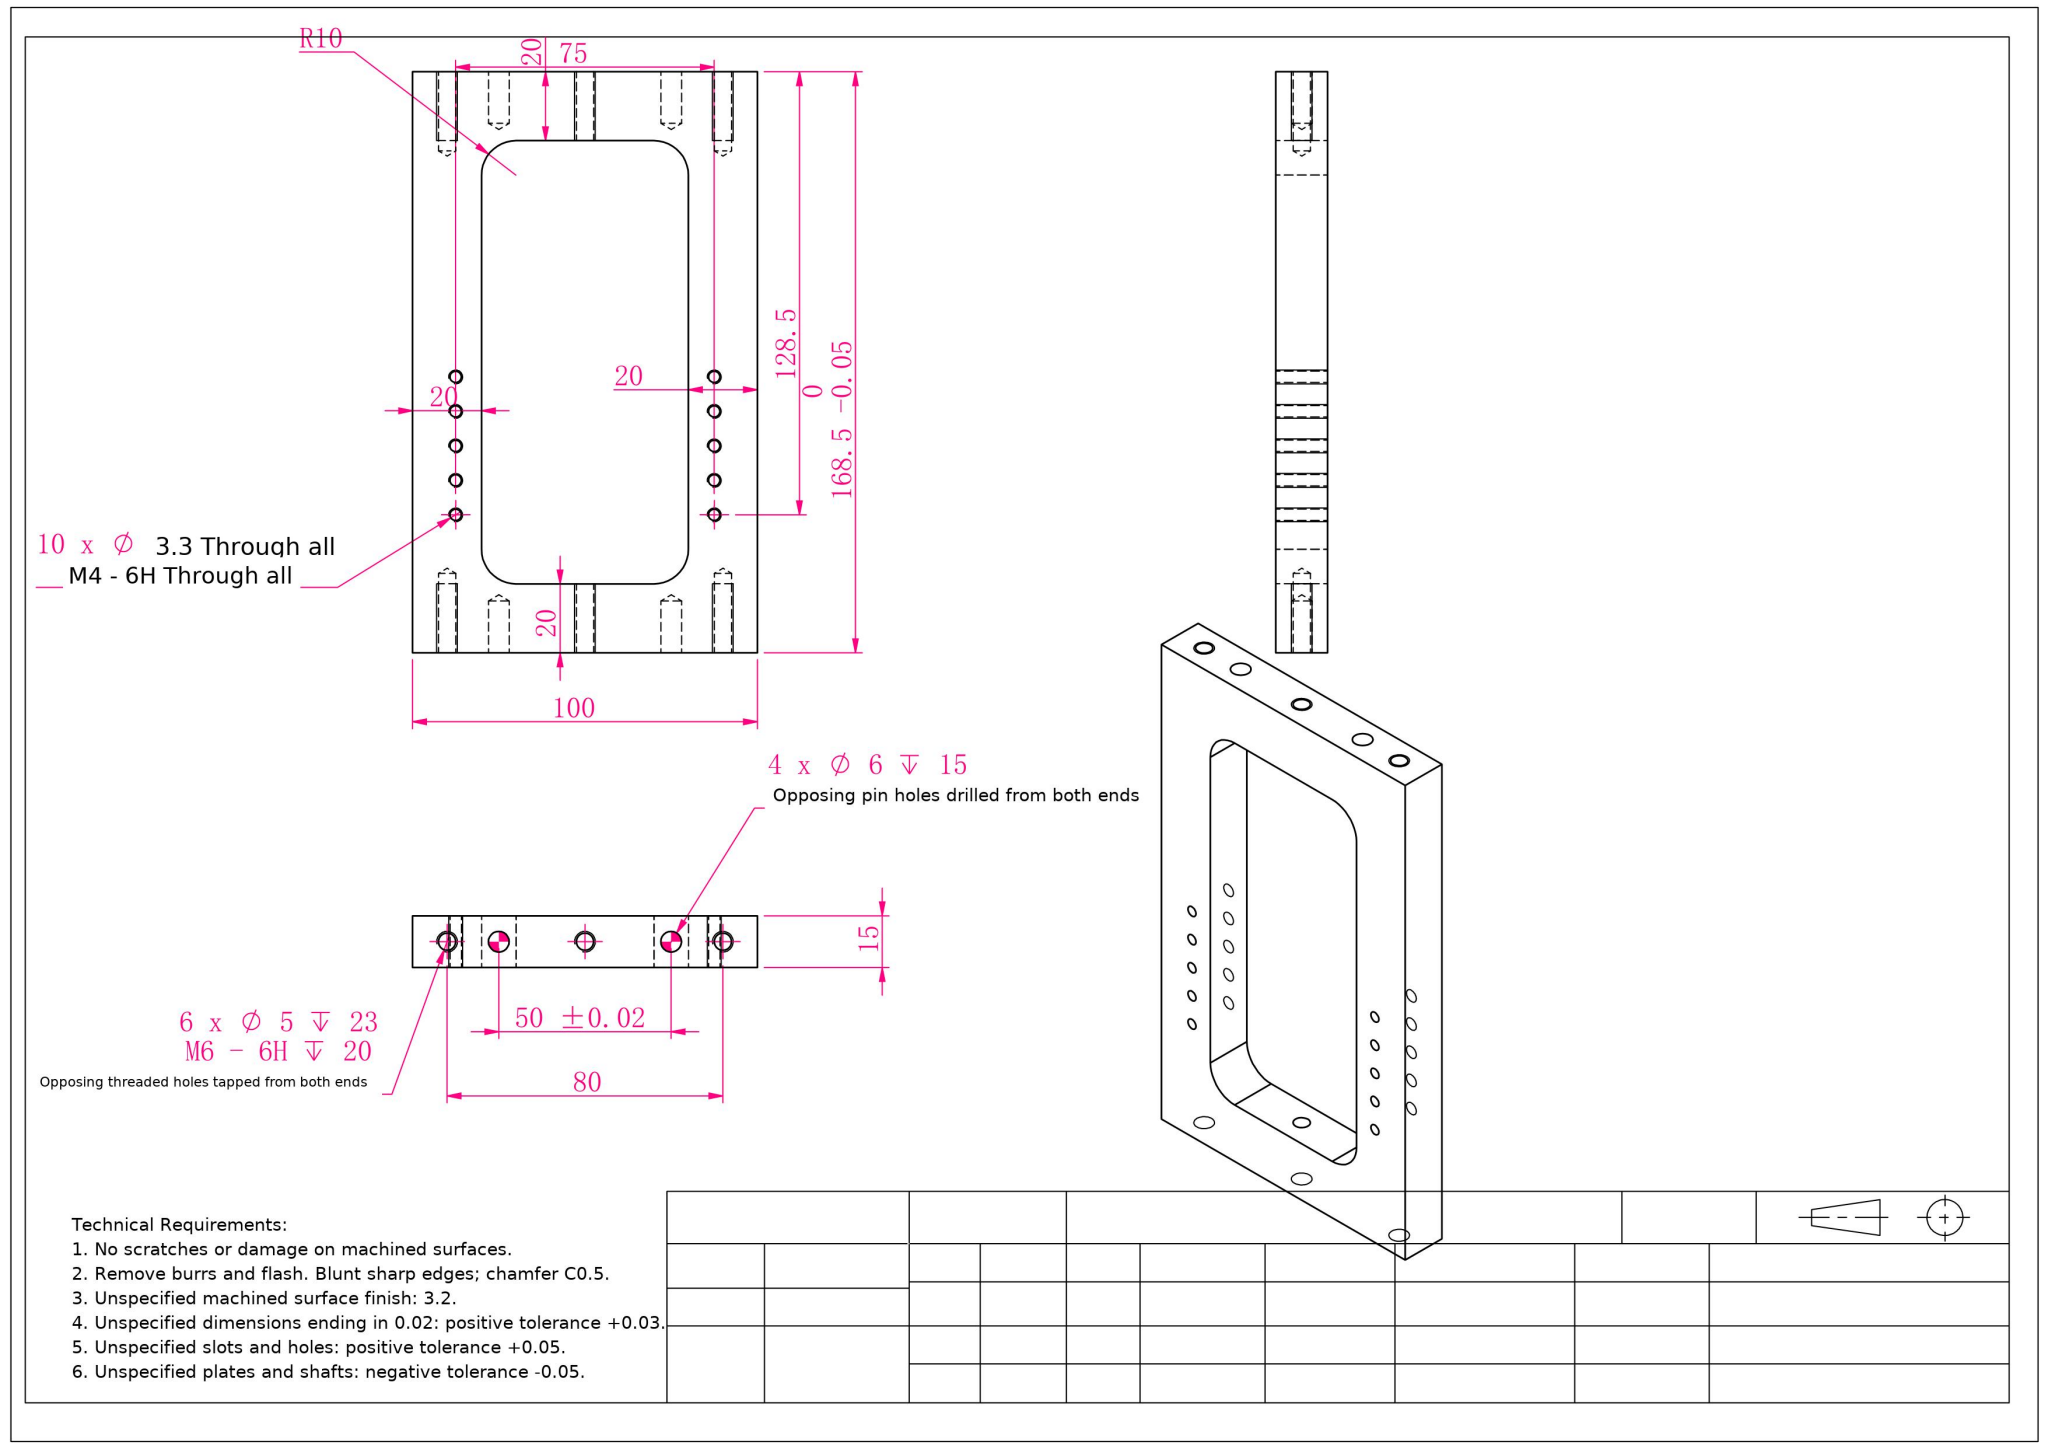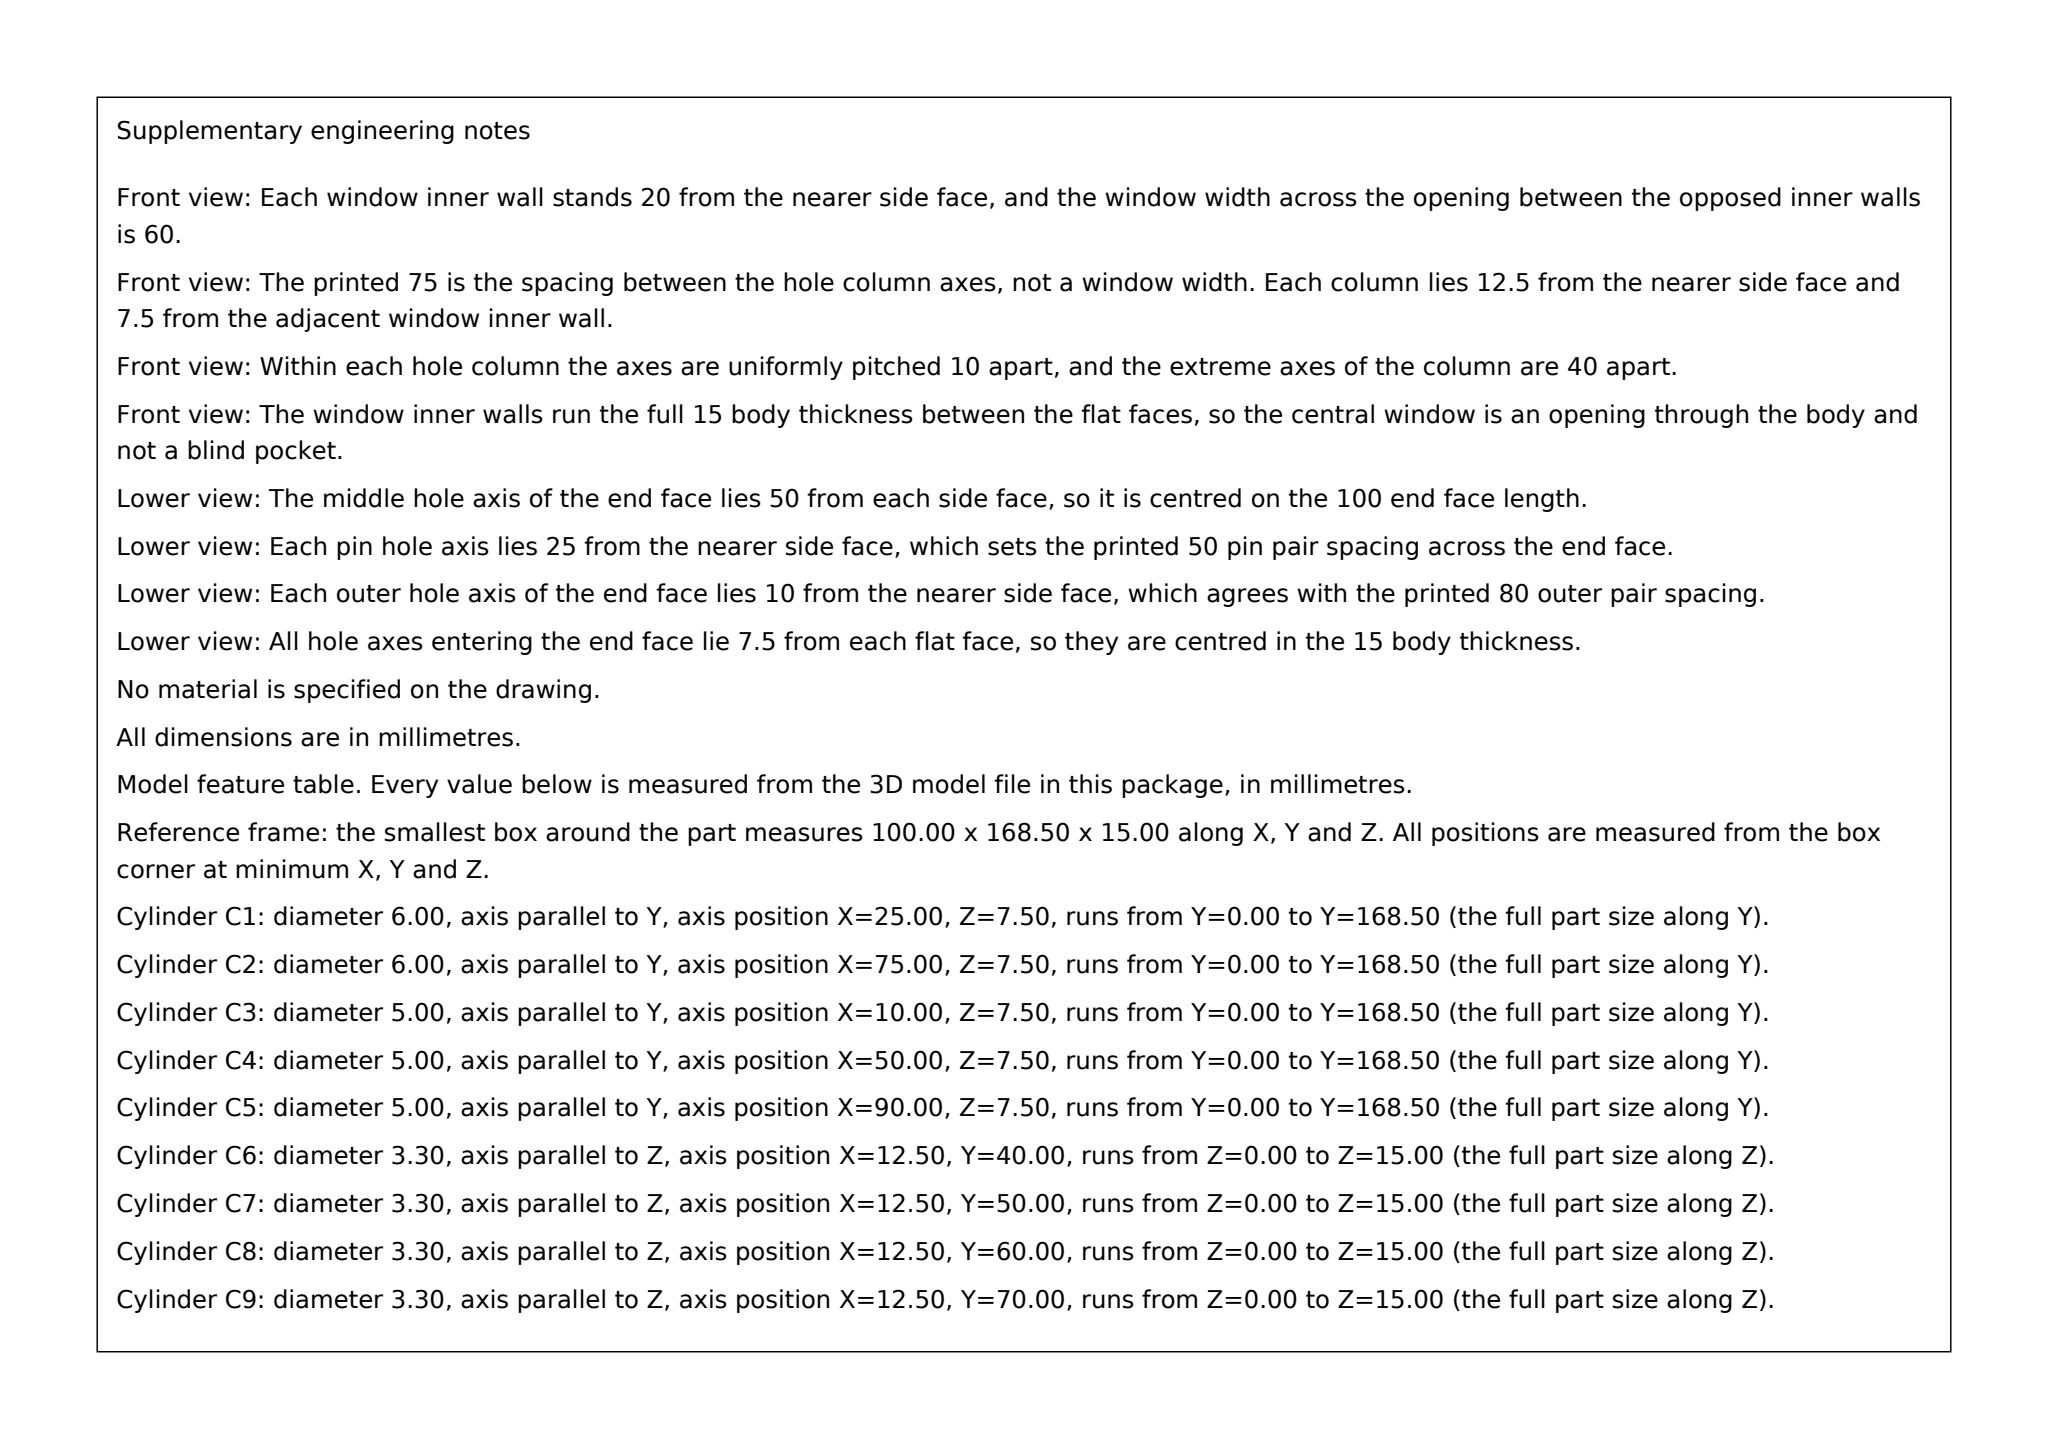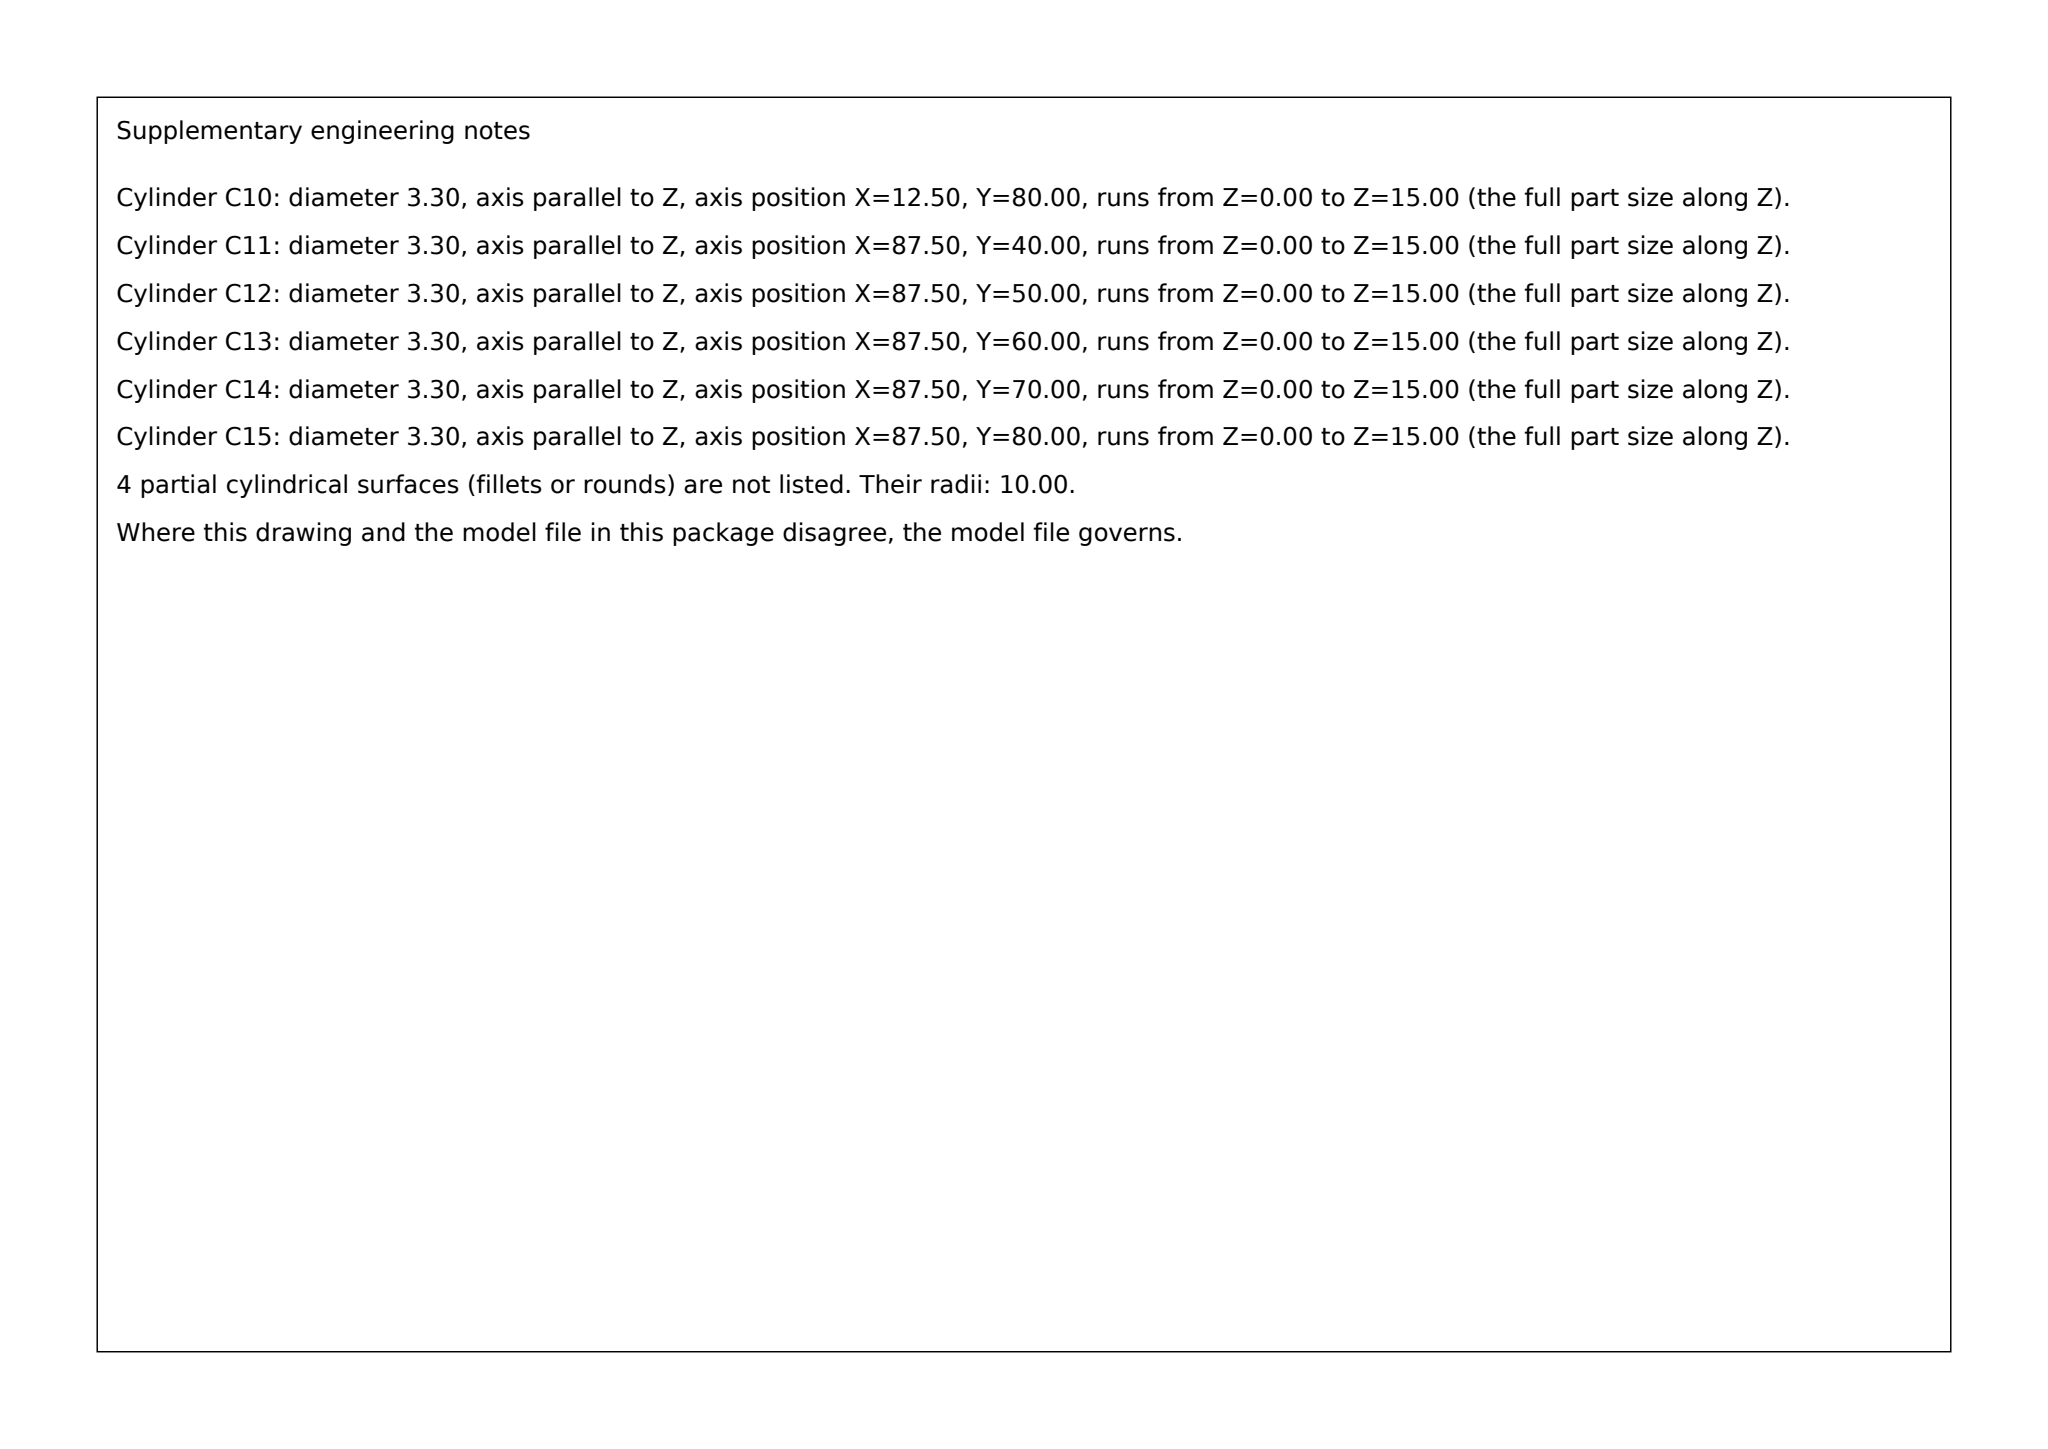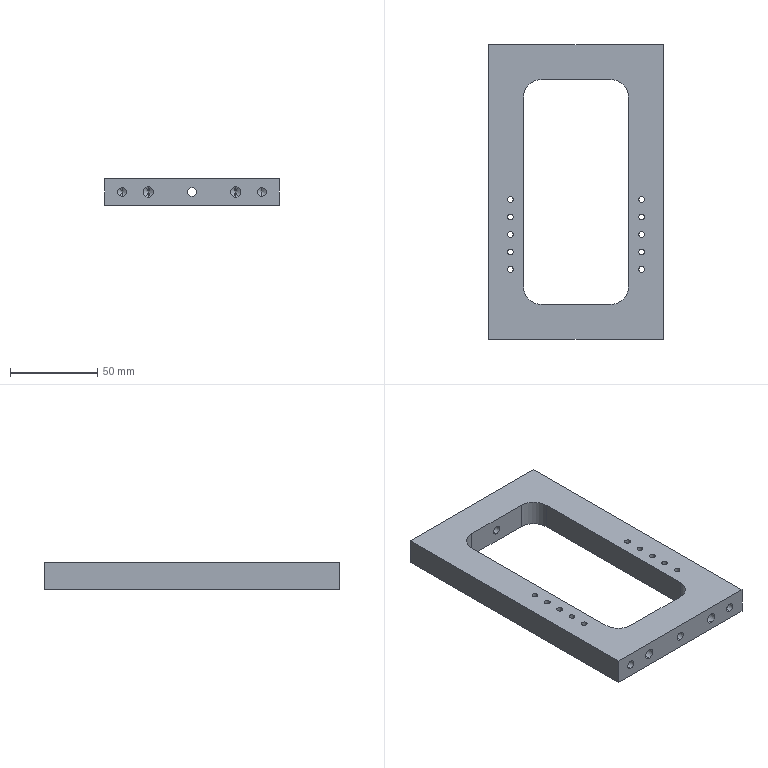Part | SolidWorks | mm | 1 solid | 70 faces | box 100 x 168.5 x 15 mm | volume 132709 mm3 | cylinder 44 | cone 16 | plane 10 | commonest cylinder face diameters 3.3 x20 5 x12 6 x8 20 x4
build123d program:
from build123d import *

# Parameters (mm, degrees)
SKETCH1_W                          = 100
SKETCH1_H                          = 168.5
BOSS_EXTRUDE1_DEPTH                = 7.5
M6_TAPPED_HOLE1_AT_2_COUNT         = 2
M6_TAPPED_HOLE1_AT_2_PITCH         = 40
M6_TAPPED_HOLE1_AT_3_COUNT         = 2
M6_TAPPED_HOLE1_AT_3_PITCH         = 80
SIZE_MM_DOWEL_PIN_HOLE1_AT_2_COUNT = 2
SIZE_MM_DOWEL_PIN_HOLE1_AT_2_PITCH = 50
SKETCH6_W                          = 60
SKETCH6_H                          = 128.5
CUT_EXTRUDE1_DEPTH                 = 100.111
FILLET1_R                          = 10
M4_TAPPED_HOLE1_D                  = 3.3
LPATTERN1_COUNT                    = 5
LPATTERN1_PITCH                    = 10


with BuildPart() as part:
    # Sketch1 → Boss-Extrude1 (new, symmetric)
    with BuildSketch(Plane.XY):
        Rectangle(SKETCH1_W, SKETCH1_H)
    extrude(amount=BOSS_EXTRUDE1_DEPTH, both=True)

    # Sketch3 → M6 Tapped Hole1 (revolve, cut)
    with BuildSketch(Plane(origin=(-40, -84.25, 0), x_dir=(0, 0, -1), z_dir=(1, 0, 0))):
        Polygon((0, 0), (0, 24.502), (2.5, 23), (2.5, 0), align=None)
    m6_tapped_hole1 = revolve(axis=Axis((-40, -90.6, 0), (0, 1, 0)), mode=Mode.SUBTRACT)

    # M6 Tapped Hole1 at 2: M6 Tapped Hole1 ×2
    with Locations(*[(i * M6_TAPPED_HOLE1_AT_2_PITCH, 0, 0) for i in range(1, M6_TAPPED_HOLE1_AT_2_COUNT)]):
        add(m6_tapped_hole1, mode=Mode.SUBTRACT)

    # M6 Tapped Hole1 at 3: M6 Tapped Hole1 ×2
    with Locations(*[(i * M6_TAPPED_HOLE1_AT_3_PITCH, 0, 0) for i in range(1, M6_TAPPED_HOLE1_AT_3_COUNT)]):
        add(m6_tapped_hole1, mode=Mode.SUBTRACT)

    # Sketch5 → Size mm Dowel Pin Hole1 (revolve, cut)
    with BuildSketch(Plane(origin=(-25, -84.25, 0), x_dir=(0, 0, -1), z_dir=(1, 0, 0))):
        Polygon((0, 0), (0, 16.803), (3, 15), (3, 0), align=None)
    size_mm_dowel_pin_hole1 = revolve(axis=Axis((-25, -90.6, 0), (0, 1, 0)), mode=Mode.SUBTRACT)

    # Size mm Dowel Pin Hole1 at 2: Size mm Dowel Pin Hole1 ×2
    with Locations(*[(i * SIZE_MM_DOWEL_PIN_HOLE1_AT_2_PITCH, 0, 0) for i in range(1, SIZE_MM_DOWEL_PIN_HOLE1_AT_2_COUNT)]):
        add(size_mm_dowel_pin_hole1, mode=Mode.SUBTRACT)

    # Mirror1: M6 Tapped Hole1, Size mm Dowel Pin Hole1 across plane
    add(m6_tapped_hole1.mirror(Plane.ZX), mode=Mode.SUBTRACT)
    add(size_mm_dowel_pin_hole1.mirror(Plane.ZX), mode=Mode.SUBTRACT)

    # Mirror1 copy 1 sketch → Mirror1 copy 1 (revolve, cut)
    with BuildSketch(Plane(origin=(0, 84.25, 0), x_dir=(0, 0, -1), z_dir=(1, 0, 0))):
        Polygon((0, 0), (0, -24.502), (2.5, -23), (2.5, 0), align=None)
    revolve(axis=Axis((0, 90.6, 0), (0, 1, 0)), mode=Mode.SUBTRACT)

    # Mirror1 copy 2 sketch → Mirror1 copy 2 (revolve, cut)
    with BuildSketch(Plane(origin=(40, 84.25, 0), x_dir=(0, 0, -1), z_dir=(1, 0, 0))):
        Polygon((0, 0), (0, -24.502), (2.5, -23), (2.5, 0), align=None)
    revolve(axis=Axis((40, 90.6, 0), (0, 1, 0)), mode=Mode.SUBTRACT)

    # Mirror1 copy 3 sketch → Mirror1 copy 3 (revolve, cut)
    with BuildSketch(Plane(origin=(25, 84.25, 0), x_dir=(0, 0, -1), z_dir=(1, 0, 0))):
        Polygon((0, 0), (0, -16.803), (3, -15), (3, 0), align=None)
    revolve(axis=Axis((25, 90.6, 0), (0, 1, 0)), mode=Mode.SUBTRACT)

    # Sketch6 → Cut-Extrude1 (cut, through all)
    with BuildSketch(Plane.XY.offset(7.5)):
        Rectangle(SKETCH6_W, SKETCH6_H)
    extrude(amount=-CUT_EXTRUDE1_DEPTH, mode=Mode.SUBTRACT)

    # Fillet1
    fillet1_edges = [part.edges().sort_by_distance(p)[0] for p in [
        (30, -64.25, 0),
        (-30, 64.25, 0),
        (30, 64.25, 0),
        (-30, -64.25, 0),
    ]]
    fillet(fillet1_edges, radius=FILLET1_R)

    # M4 Tapped Hole1 (through all)
    with Locations(Plane(origin=(0, 0, -7.5), x_dir=(-1, 0, 0), z_dir=(0, 0, -1))):
        with Locations((-37.5, -44.25), (37.5, -44.25)):
            m4_tapped_hole1 = Hole(M4_TAPPED_HOLE1_D / 2)

    # LPattern1: M4 Tapped Hole1 ×5
    with Locations(*[(0, i * LPATTERN1_PITCH, 0) for i in range(1, LPATTERN1_COUNT)]):
        add(m4_tapped_hole1, mode=Mode.SUBTRACT)


solid = part.part